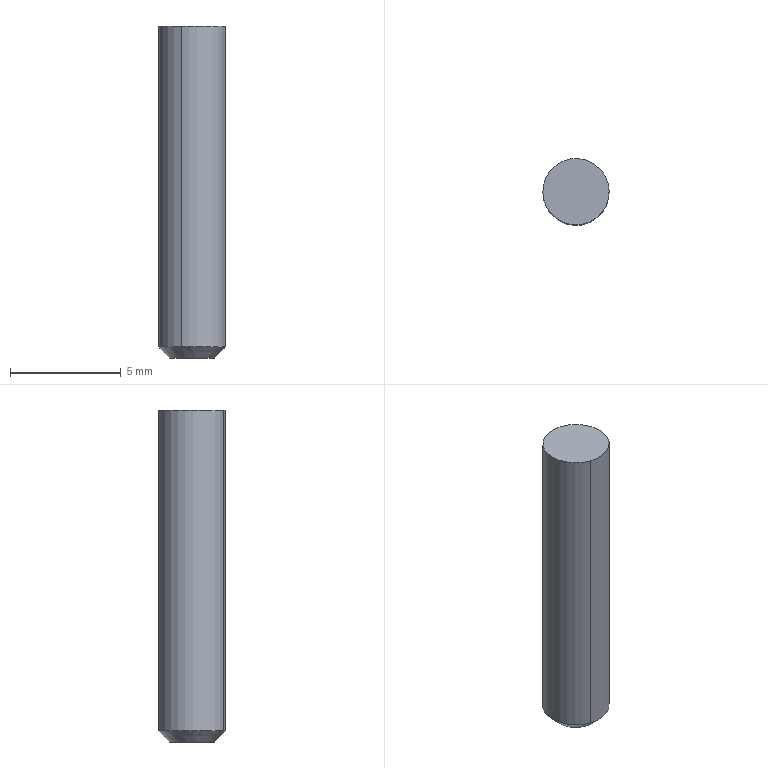Component | SolidWorks | GB-T15389-1994-M3-20StudNew-1 | 1 solid | 6 faces | box 3 x 3 x 15 mm | volume 105 mm3 | cone 2 | cylinder 2 | plane 2 | commonest cylinder face diameters 3 x2
build123d program:
from build123d import *

# Parameters (mm, degrees)
SKETCH1_R           = 1.5
BOSS_EXTRUDE1_DEPTH = 15
CHAMFER1_SIZE       = 0.5


with BuildPart() as part:
    # Sketch1 → Boss-Extrude1 (new body)
    with BuildSketch(Plane(origin=(0, 0, 0), x_dir=(1, 0, 0), z_dir=(0, 1, 0))):
        with Locations(Location((0, 0, 0), (0, 0, 270))):
            Circle(SKETCH1_R)
    extrude(amount=BOSS_EXTRUDE1_DEPTH)

    # Chamfer1
    chamfer1_edges = [part.edges().sort_by_distance(p)[0] for p in [
        (0, 15, -1.5),
    ]]
    chamfer(chamfer1_edges, length=CHAMFER1_SIZE)


solid = part.part

# Placed as in the assembly
solid = solid.moved(Location((1240.186, 993.812, 1434.454), (-90, 0, 0)))
STEP:
#1=CARTESIAN_POINT('',(48.814,39.089,55.884));
#2=VERTEX_POINT('',#1);
#3=CARTESIAN_POINT('',(48.839,39.164,55.884));
#4=VERTEX_POINT('',#3);
#5=CARTESIAN_POINT('',(48.826,39.126,55.884));
#6=DIRECTION('',(-0.,0.,-1.));
#7=DIRECTION('',(-0.316,-0.9488,0.));
#8=AXIS2_PLACEMENT_3D('',#5,#6,#7);
#9=CIRCLE('',#8,0.03937);
#10=EDGE_CURVE('',#2,#4,#9,.T.);
#11=ORIENTED_EDGE('',*,*,#10,.F.);
#12=CARTESIAN_POINT('',(48.808,39.07,55.904));
#13=VERTEX_POINT('',#12);
#14=CARTESIAN_POINT('',(48.814,39.089,55.884));
#15=DIRECTION('',(-0.2235,-0.6709,0.7071));
#16=VECTOR('',#15,39.37);
#17=LINE('',#14,#16);
#18=EDGE_CURVE('',#2,#13,#17,.T.);
#19=ORIENTED_EDGE('',*,*,#18,.T.);
#20=CARTESIAN_POINT('',(48.845,39.182,55.904));
#21=VERTEX_POINT('',#20);
#22=CARTESIAN_POINT('',(48.826,39.126,55.904));
#23=DIRECTION('',(0.,-0.,1.));
#24=DIRECTION('',(-0.316,-0.9488,0.));
#25=AXIS2_PLACEMENT_3D('',#22,#23,#24);
#26=CIRCLE('',#25,0.05906);
#27=EDGE_CURVE('',#21,#13,#26,.T.);
#28=ORIENTED_EDGE('',*,*,#27,.F.);
#29=CARTESIAN_POINT('',(48.839,39.164,55.884));
#30=DIRECTION('',(0.2235,0.6709,0.7071));
#31=VECTOR('',#30,39.37);
#32=LINE('',#29,#31);
#33=EDGE_CURVE('',#4,#21,#32,.T.);
#34=ORIENTED_EDGE('',*,*,#33,.F.);
#35=EDGE_LOOP('',(#11,#19,#28,#34));
#36=FACE_OUTER_BOUND('',#35,.T.);
#37=CARTESIAN_POINT('',(48.826,39.126,55.884));
#38=DIRECTION('',(0.,-0.,1.));
#39=DIRECTION('',(0.316,0.9488,0.));
#40=AXIS2_PLACEMENT_3D('',#37,#38,#39);
#41=CONICAL_SURFACE('',#40,0.03937,0.7854);
#42=ADVANCED_FACE('',(#36),#41,.T.);
#43=ORIENTED_EDGE('',*,*,#27,.T.);
#44=CARTESIAN_POINT('',(48.808,39.07,56.475));
#45=VERTEX_POINT('',#44);
#46=CARTESIAN_POINT('',(48.808,39.07,55.884));
#47=DIRECTION('',(0.,-0.,1.));
#48=VECTOR('',#47,39.37);
#49=LINE('',#46,#48);
#50=EDGE_CURVE('',#13,#45,#49,.T.);
#51=ORIENTED_EDGE('',*,*,#50,.T.);
#52=CARTESIAN_POINT('',(48.845,39.182,56.475));
#53=VERTEX_POINT('',#52);
#54=CARTESIAN_POINT('',(48.826,39.126,56.475));
#55=DIRECTION('',(-0.,0.,-1.));
#56=DIRECTION('',(-0.316,-0.9488,0.));
#57=AXIS2_PLACEMENT_3D('',#54,#55,#56);
#58=CIRCLE('',#57,0.05906);
#59=EDGE_CURVE('',#45,#53,#58,.T.);
#60=ORIENTED_EDGE('',*,*,#59,.T.);
#61=CARTESIAN_POINT('',(48.845,39.182,55.884));
#62=DIRECTION('',(0.,-0.,1.));
#63=VECTOR('',#62,39.37);
#64=LINE('',#61,#63);
#65=EDGE_CURVE('',#21,#53,#64,.T.);
#66=ORIENTED_EDGE('',*,*,#65,.F.);
#67=EDGE_LOOP('',(#43,#51,#60,#66));
#68=FACE_OUTER_BOUND('',#67,.T.);
#69=CARTESIAN_POINT('',(48.826,39.126,55.884));
#70=DIRECTION('',(0.,-0.,1.));
#71=DIRECTION('',(0.316,0.9488,0.));
#72=AXIS2_PLACEMENT_3D('',#69,#70,#71);
#73=CYLINDRICAL_SURFACE('',#72,0.05906);
#74=ADVANCED_FACE('',(#68),#73,.T.);
#75=ORIENTED_EDGE('',*,*,#50,.F.);
#76=CARTESIAN_POINT('',(48.826,39.126,55.904));
#77=DIRECTION('',(0.,-0.,1.));
#78=DIRECTION('',(-0.316,-0.9488,0.));
#79=AXIS2_PLACEMENT_3D('',#76,#77,#78);
#80=CIRCLE('',#79,0.05906);
#81=EDGE_CURVE('',#13,#21,#80,.T.);
#82=ORIENTED_EDGE('',*,*,#81,.T.);
#83=ORIENTED_EDGE('',*,*,#65,.T.);
#84=CARTESIAN_POINT('',(48.826,39.126,56.475));
#85=DIRECTION('',(-0.,0.,-1.));
#86=DIRECTION('',(-0.316,-0.9488,0.));
#87=AXIS2_PLACEMENT_3D('',#84,#85,#86);
#88=CIRCLE('',#87,0.05906);
#89=EDGE_CURVE('',#53,#45,#88,.T.);
#90=ORIENTED_EDGE('',*,*,#89,.T.);
#91=EDGE_LOOP('',(#75,#82,#83,#90));
#92=FACE_OUTER_BOUND('',#91,.T.);
#93=CARTESIAN_POINT('',(48.826,39.126,55.884));
#94=DIRECTION('',(0.,-0.,1.));
#95=DIRECTION('',(0.316,0.9488,0.));
#96=AXIS2_PLACEMENT_3D('',#93,#94,#95);
#97=CYLINDRICAL_SURFACE('',#96,0.05906);
#98=ADVANCED_FACE('',(#92),#97,.T.);
#99=CARTESIAN_POINT('',(48.826,39.126,55.884));
#100=DIRECTION('',(-0.,0.,-1.));
#101=DIRECTION('',(-0.316,-0.9488,0.));
#102=AXIS2_PLACEMENT_3D('',#99,#100,#101);
#103=CIRCLE('',#102,0.03937);
#104=EDGE_CURVE('',#4,#2,#103,.T.);
#105=ORIENTED_EDGE('',*,*,#104,.T.);
#106=ORIENTED_EDGE('',*,*,#10,.T.);
#107=EDGE_LOOP('',(#105,#106));
#108=FACE_OUTER_BOUND('',#107,.T.);
#109=CARTESIAN_POINT('',(48.826,39.126,55.884));
#110=DIRECTION('',(-0.,0.,-1.));
#111=DIRECTION('',(-0.316,-0.9488,-0.));
#112=AXIS2_PLACEMENT_3D('',#109,#110,#111);
#113=PLANE('',#112);
#114=ADVANCED_FACE('',(#108),#113,.T.);
#115=ORIENTED_EDGE('',*,*,#89,.F.);
#116=ORIENTED_EDGE('',*,*,#59,.F.);
#117=EDGE_LOOP('',(#115,#116));
#118=FACE_OUTER_BOUND('',#117,.T.);
#119=CARTESIAN_POINT('',(48.826,39.126,56.475));
#120=DIRECTION('',(-0.,0.,-1.));
#121=DIRECTION('',(-0.316,-0.9488,-0.));
#122=AXIS2_PLACEMENT_3D('',#119,#120,#121);
#123=PLANE('',#122);
#124=ADVANCED_FACE('',(#118),#123,.F.);
#125=ORIENTED_EDGE('',*,*,#18,.F.);
#126=ORIENTED_EDGE('',*,*,#104,.F.);
#127=ORIENTED_EDGE('',*,*,#33,.T.);
#128=ORIENTED_EDGE('',*,*,#81,.F.);
#129=EDGE_LOOP('',(#125,#126,#127,#128));
#130=FACE_OUTER_BOUND('',#129,.T.);
#131=CARTESIAN_POINT('',(48.826,39.126,55.884));
#132=DIRECTION('',(0.,-0.,1.));
#133=DIRECTION('',(0.316,0.9488,0.));
#134=AXIS2_PLACEMENT_3D('',#131,#132,#133);
#135=CONICAL_SURFACE('',#134,0.03937,0.7854);
#136=ADVANCED_FACE('',(#130),#135,.T.);
#137=CLOSED_SHELL('',(#42,#74,#98,#114,#124,#136));
#138=MANIFOLD_SOLID_BREP('',#137);
#139=CARTESIAN_POINT('',(0.,0.,0.));
#140=DIRECTION('',(0.,0.,1.));
#141=DIRECTION('',(1.,0.,0.));
#142=AXIS2_PLACEMENT_3D('',#139,#140,#141);
#143=(LENGTH_UNIT()NAMED_UNIT(*)SI_UNIT($,.METRE.));
#144=LENGTH_MEASURE_WITH_UNIT(LENGTH_MEASURE(0.0254),#143);
#145=DIMENSIONAL_EXPONENTS(1.,0.,0.,0.,0.,0.,0.);
#146=(CONVERSION_BASED_UNIT('',#144)LENGTH_UNIT()NAMED_UNIT(#145));
#147=UNCERTAINTY_MEASURE_WITH_UNIT(LENGTH_MEASURE(0.00001),#146,'','');
#148=(NAMED_UNIT(*)PLANE_ANGLE_UNIT()SI_UNIT($,.RADIAN.));
#149=(NAMED_UNIT(*)SI_UNIT($,.STERADIAN.)SOLID_ANGLE_UNIT());
#150=(GEOMETRIC_REPRESENTATION_CONTEXT(3)GLOBAL_UNCERTAINTY_ASSIGNED_CONTEXT((#147))GLOBAL_UNIT_ASSIGNED_CONTEXT((#146,#148,#149))REPRESENTATION_CONTEXT('',''));
#151=ADVANCED_BREP_SHAPE_REPRESENTATION('',(#138,#142),#150);
#152=COLOUR_RGB('',0.7922,0.8196,0.9333);
#153=FILL_AREA_STYLE_COLOUR('',#152);
#154=FILL_AREA_STYLE('',(#153));
#155=SURFACE_STYLE_FILL_AREA(#154);
#156=SURFACE_SIDE_STYLE('',(#155));
#157=SURFACE_STYLE_USAGE(.BOTH.,#156);
#158=PRESENTATION_STYLE_ASSIGNMENT((#157));
#159=STYLED_ITEM('',(#158),#138);
#160=(LENGTH_UNIT()NAMED_UNIT(*)SI_UNIT($,.METRE.));
#161=LENGTH_MEASURE_WITH_UNIT(LENGTH_MEASURE(0.0254),#160);
#162=DIMENSIONAL_EXPONENTS(1.,0.,0.,0.,0.,0.,0.);
#163=(CONVERSION_BASED_UNIT('',#161)LENGTH_UNIT()NAMED_UNIT(#162));
#164=UNCERTAINTY_MEASURE_WITH_UNIT(LENGTH_MEASURE(0.00001),#163,'','');
#165=(NAMED_UNIT(*)PLANE_ANGLE_UNIT()SI_UNIT($,.RADIAN.));
#166=(NAMED_UNIT(*)SI_UNIT($,.STERADIAN.)SOLID_ANGLE_UNIT());
#167=(GEOMETRIC_REPRESENTATION_CONTEXT(3)GLOBAL_UNCERTAINTY_ASSIGNED_CONTEXT((#164))GLOBAL_UNIT_ASSIGNED_CONTEXT((#163,#165,#166))REPRESENTATION_CONTEXT('',''));
#168=MECHANICAL_DESIGN_GEOMETRIC_PRESENTATION_REPRESENTATION('',(#159),#167);
#169=PRESENTATION_LAYER_ASSIGNMENT('','',(#159));